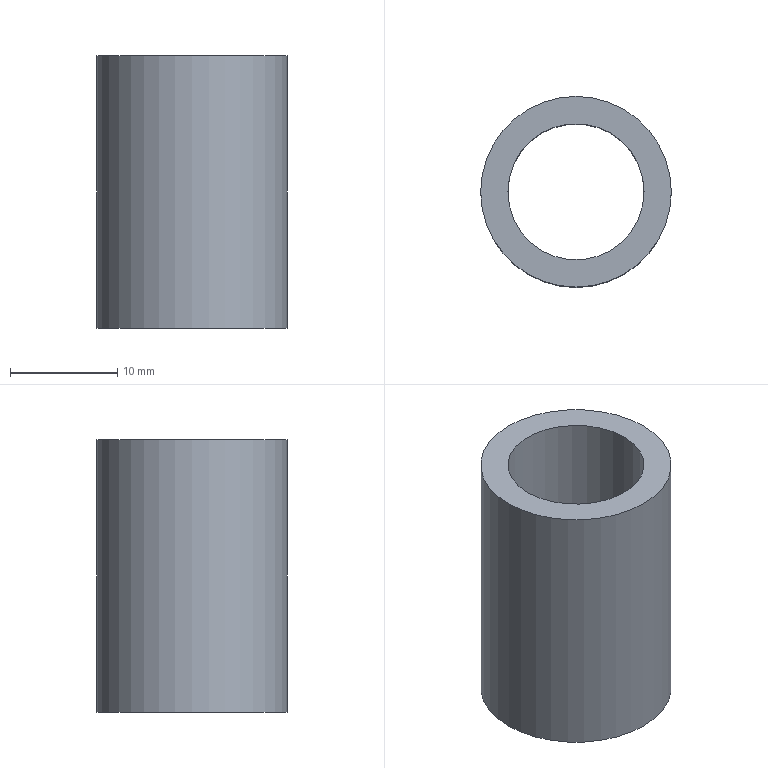Component | NX | SLEEVE | 1 solid | 4 faces | box 17.78 x 17.78 x 25.4 mm | volume 3089 mm3 | cylinder 2 | plane 2 | commonest cylinder face diameters 17.78 x1 12.7 x1
STEP:
#1=CARTESIAN_POINT('',(0.,0.,0.));
#2=DIRECTION('',(0.,0.,1.));
#3=DIRECTION('',(1.,0.,0.));
#4=AXIS2_PLACEMENT_3D('',#1,#2,#3);
#5=CARTESIAN_POINT('',(8.89,0.,627.));
#6=VERTEX_POINT('',#5);
#7=CARTESIAN_POINT('',(0.,0.,627.));
#8=DIRECTION('',(0.,0.,1.));
#9=DIRECTION('',(1.,0.,0.));
#10=AXIS2_PLACEMENT_3D('',#7,#8,#9);
#11=CIRCLE('',#10,8.89);
#12=CARTESIAN_POINT('',(0.,0.,627.));
#13=DIRECTION('',(0.,0.,-1.));
#14=DIRECTION('',(-1.,0.,0.));
#15=AXIS2_PLACEMENT_3D('',#12,#13,#14);
#16=CYLINDRICAL_SURFACE('',#15,8.89);
#17=CARTESIAN_POINT('',(9.425,0.));
#18=DIRECTION('',(-1.,0.));
#19=VECTOR('',#18,1.);
#20=LINE('',#17,#19);
#21=(GEOMETRIC_REPRESENTATION_CONTEXT(2)PARAMETRIC_REPRESENTATION_CONTEXT()REPRESENTATION_CONTEXT('',''));
#22=DEFINITIONAL_REPRESENTATION('',(#20),#21);
#23=PCURVE('',#16,#22);
#24=CARTESIAN_POINT('',(0.,0.,627.));
#25=DIRECTION('',(0.,0.,1.));
#26=DIRECTION('',(1.,0.,0.));
#27=AXIS2_PLACEMENT_3D('',#24,#25,#26);
#28=PLANE('',#27);
#29=CARTESIAN_POINT('',(0.,0.));
#30=DIRECTION('',(1.,0.));
#31=AXIS2_PLACEMENT_2D('',#29,#30);
#32=CIRCLE('',#31,8.89);
#33=(GEOMETRIC_REPRESENTATION_CONTEXT(2)PARAMETRIC_REPRESENTATION_CONTEXT()REPRESENTATION_CONTEXT('',''));
#34=DEFINITIONAL_REPRESENTATION('',(#32),#33);
#35=PCURVE('',#28,#34);
#36=SURFACE_CURVE('',#11,(#23,#35),.PCURVE_S1.);
#37=EDGE_CURVE('',#6,#6,#36,.T.);
#38=ORIENTED_EDGE('',*,*,#37,.F.);
#39=CARTESIAN_POINT('',(8.89,0.,601.6));
#40=VERTEX_POINT('',#39);
#41=CARTESIAN_POINT('',(8.89,0.,627.));
#42=CARTESIAN_POINT('',(8.89,0.,601.6));
#43=B_SPLINE_CURVE_WITH_KNOTS('',1,(#41,#42),.UNSPECIFIED.,.F.,.F.,(2,2),(0.,25.4),.PIECEWISE_BEZIER_KNOTS.);
#44=CARTESIAN_POINT('',(9.425,0.));
#45=DIRECTION('',(0.,1.));
#46=VECTOR('',#45,1.);
#47=LINE('',#44,#46);
#48=(GEOMETRIC_REPRESENTATION_CONTEXT(2)PARAMETRIC_REPRESENTATION_CONTEXT()REPRESENTATION_CONTEXT('',''));
#49=DEFINITIONAL_REPRESENTATION('',(#47),#48);
#50=PCURVE('',#16,#49);
#51=CARTESIAN_POINT('',(3.142,0.));
#52=DIRECTION('',(0.,1.));
#53=VECTOR('',#52,1.);
#54=LINE('',#51,#53);
#55=(GEOMETRIC_REPRESENTATION_CONTEXT(2)PARAMETRIC_REPRESENTATION_CONTEXT()REPRESENTATION_CONTEXT('',''));
#56=DEFINITIONAL_REPRESENTATION('',(#54),#55);
#57=PCURVE('',#16,#56);
#58=SEAM_CURVE('',#43,(#50,#57),.PCURVE_S1.);
#59=EDGE_CURVE('',#6,#40,#58,.T.);
#60=ORIENTED_EDGE('',*,*,#59,.T.);
#61=CARTESIAN_POINT('',(0.,0.,601.6));
#62=DIRECTION('',(0.,0.,1.));
#63=DIRECTION('',(1.,0.,0.));
#64=AXIS2_PLACEMENT_3D('',#61,#62,#63);
#65=CIRCLE('',#64,8.89);
#66=CARTESIAN_POINT('',(9.425,25.4));
#67=DIRECTION('',(-1.,0.));
#68=VECTOR('',#67,1.);
#69=LINE('',#66,#68);
#70=(GEOMETRIC_REPRESENTATION_CONTEXT(2)PARAMETRIC_REPRESENTATION_CONTEXT()REPRESENTATION_CONTEXT('',''));
#71=DEFINITIONAL_REPRESENTATION('',(#69),#70);
#72=PCURVE('',#16,#71);
#73=CARTESIAN_POINT('',(0.,0.,601.6));
#74=DIRECTION('',(0.,0.,1.));
#75=DIRECTION('',(1.,0.,0.));
#76=AXIS2_PLACEMENT_3D('',#73,#74,#75);
#77=PLANE('',#76);
#78=CARTESIAN_POINT('',(0.,0.));
#79=DIRECTION('',(1.,0.));
#80=AXIS2_PLACEMENT_2D('',#78,#79);
#81=CIRCLE('',#80,8.89);
#82=(GEOMETRIC_REPRESENTATION_CONTEXT(2)PARAMETRIC_REPRESENTATION_CONTEXT()REPRESENTATION_CONTEXT('',''));
#83=DEFINITIONAL_REPRESENTATION('',(#81),#82);
#84=PCURVE('',#77,#83);
#85=SURFACE_CURVE('',#65,(#72,#84),.PCURVE_S1.);
#86=EDGE_CURVE('',#40,#40,#85,.T.);
#87=ORIENTED_EDGE('',*,*,#86,.T.);
#88=ORIENTED_EDGE('',*,*,#59,.F.);
#89=EDGE_LOOP('',(#38,#60,#87,#88));
#90=FACE_BOUND('',#89,.T.);
#91=ADVANCED_FACE('',(#90),#16,.T.);
#92=CARTESIAN_POINT('',(6.35,0.,627.));
#93=VERTEX_POINT('',#92);
#94=CARTESIAN_POINT('',(0.,0.,627.));
#95=DIRECTION('',(0.,0.,1.));
#96=DIRECTION('',(1.,0.,0.));
#97=AXIS2_PLACEMENT_3D('',#94,#95,#96);
#98=CIRCLE('',#97,6.35);
#99=CARTESIAN_POINT('',(0.,0.,627.));
#100=DIRECTION('',(0.,0.,-1.));
#101=DIRECTION('',(-1.,0.,0.));
#102=AXIS2_PLACEMENT_3D('',#99,#100,#101);
#103=CYLINDRICAL_SURFACE('',#102,6.35);
#104=CARTESIAN_POINT('',(9.425,0.));
#105=DIRECTION('',(-1.,0.));
#106=VECTOR('',#105,1.);
#107=LINE('',#104,#106);
#108=(GEOMETRIC_REPRESENTATION_CONTEXT(2)PARAMETRIC_REPRESENTATION_CONTEXT()REPRESENTATION_CONTEXT('',''));
#109=DEFINITIONAL_REPRESENTATION('',(#107),#108);
#110=PCURVE('',#103,#109);
#111=CARTESIAN_POINT('',(0.,0.));
#112=DIRECTION('',(1.,0.));
#113=AXIS2_PLACEMENT_2D('',#111,#112);
#114=CIRCLE('',#113,6.35);
#115=(GEOMETRIC_REPRESENTATION_CONTEXT(2)PARAMETRIC_REPRESENTATION_CONTEXT()REPRESENTATION_CONTEXT('',''));
#116=DEFINITIONAL_REPRESENTATION('',(#114),#115);
#117=PCURVE('',#28,#116);
#118=SURFACE_CURVE('',#98,(#110,#117),.PCURVE_S1.);
#119=EDGE_CURVE('',#93,#93,#118,.T.);
#120=ORIENTED_EDGE('',*,*,#119,.F.);
#121=CARTESIAN_POINT('',(6.35,0.,601.6));
#122=VERTEX_POINT('',#121);
#123=CARTESIAN_POINT('',(6.35,0.,627.));
#124=CARTESIAN_POINT('',(6.35,0.,601.6));
#125=B_SPLINE_CURVE_WITH_KNOTS('',1,(#123,#124),.UNSPECIFIED.,.F.,.F.,(2,2),(0.,25.4),.PIECEWISE_BEZIER_KNOTS.);
#126=CARTESIAN_POINT('',(9.425,0.));
#127=DIRECTION('',(0.,1.));
#128=VECTOR('',#127,1.);
#129=LINE('',#126,#128);
#130=(GEOMETRIC_REPRESENTATION_CONTEXT(2)PARAMETRIC_REPRESENTATION_CONTEXT()REPRESENTATION_CONTEXT('',''));
#131=DEFINITIONAL_REPRESENTATION('',(#129),#130);
#132=PCURVE('',#103,#131);
#133=CARTESIAN_POINT('',(3.142,0.));
#134=DIRECTION('',(0.,1.));
#135=VECTOR('',#134,1.);
#136=LINE('',#133,#135);
#137=(GEOMETRIC_REPRESENTATION_CONTEXT(2)PARAMETRIC_REPRESENTATION_CONTEXT()REPRESENTATION_CONTEXT('',''));
#138=DEFINITIONAL_REPRESENTATION('',(#136),#137);
#139=PCURVE('',#103,#138);
#140=SEAM_CURVE('',#125,(#132,#139),.PCURVE_S1.);
#141=EDGE_CURVE('',#93,#122,#140,.T.);
#142=ORIENTED_EDGE('',*,*,#141,.T.);
#143=CARTESIAN_POINT('',(0.,0.,601.6));
#144=DIRECTION('',(0.,0.,1.));
#145=DIRECTION('',(1.,0.,0.));
#146=AXIS2_PLACEMENT_3D('',#143,#144,#145);
#147=CIRCLE('',#146,6.35);
#148=CARTESIAN_POINT('',(9.425,25.4));
#149=DIRECTION('',(-1.,0.));
#150=VECTOR('',#149,1.);
#151=LINE('',#148,#150);
#152=(GEOMETRIC_REPRESENTATION_CONTEXT(2)PARAMETRIC_REPRESENTATION_CONTEXT()REPRESENTATION_CONTEXT('',''));
#153=DEFINITIONAL_REPRESENTATION('',(#151),#152);
#154=PCURVE('',#103,#153);
#155=CARTESIAN_POINT('',(0.,0.));
#156=DIRECTION('',(1.,0.));
#157=AXIS2_PLACEMENT_2D('',#155,#156);
#158=CIRCLE('',#157,6.35);
#159=(GEOMETRIC_REPRESENTATION_CONTEXT(2)PARAMETRIC_REPRESENTATION_CONTEXT()REPRESENTATION_CONTEXT('',''));
#160=DEFINITIONAL_REPRESENTATION('',(#158),#159);
#161=PCURVE('',#77,#160);
#162=SURFACE_CURVE('',#147,(#154,#161),.PCURVE_S1.);
#163=EDGE_CURVE('',#122,#122,#162,.T.);
#164=ORIENTED_EDGE('',*,*,#163,.T.);
#165=ORIENTED_EDGE('',*,*,#141,.F.);
#166=EDGE_LOOP('',(#120,#142,#164,#165));
#167=FACE_BOUND('',#166,.F.);
#168=ADVANCED_FACE('',(#167),#103,.F.);
#169=ORIENTED_EDGE('',*,*,#37,.T.);
#170=EDGE_LOOP('',(#169));
#171=FACE_BOUND('',#170,.T.);
#172=ORIENTED_EDGE('',*,*,#119,.F.);
#173=EDGE_LOOP('',(#172));
#174=FACE_BOUND('',#173,.T.);
#175=ADVANCED_FACE('',(#171,#174),#28,.T.);
#176=ORIENTED_EDGE('',*,*,#86,.F.);
#177=EDGE_LOOP('',(#176));
#178=FACE_BOUND('',#177,.T.);
#179=ORIENTED_EDGE('',*,*,#163,.T.);
#180=EDGE_LOOP('',(#179));
#181=FACE_BOUND('',#180,.T.);
#182=ADVANCED_FACE('',(#178,#181),#77,.F.);
#183=CLOSED_SHELL('',(#91,#168,#175,#182));
#184=MANIFOLD_SOLID_BREP('',#183);
#185=(LENGTH_UNIT()NAMED_UNIT(*)SI_UNIT(.MILLI.,.METRE.));
#186=UNCERTAINTY_MEASURE_WITH_UNIT(LENGTH_MEASURE(0.00001),#185,'','');
#187=(NAMED_UNIT(*)PLANE_ANGLE_UNIT()SI_UNIT($,.RADIAN.));
#188=(NAMED_UNIT(*)SI_UNIT($,.STERADIAN.)SOLID_ANGLE_UNIT());
#189=(GEOMETRIC_REPRESENTATION_CONTEXT(3)GLOBAL_UNCERTAINTY_ASSIGNED_CONTEXT((#186))GLOBAL_UNIT_ASSIGNED_CONTEXT((#185,#187,#188))REPRESENTATION_CONTEXT('',''));
#190=ADVANCED_BREP_SHAPE_REPRESENTATION('',(#4,#184),#189);